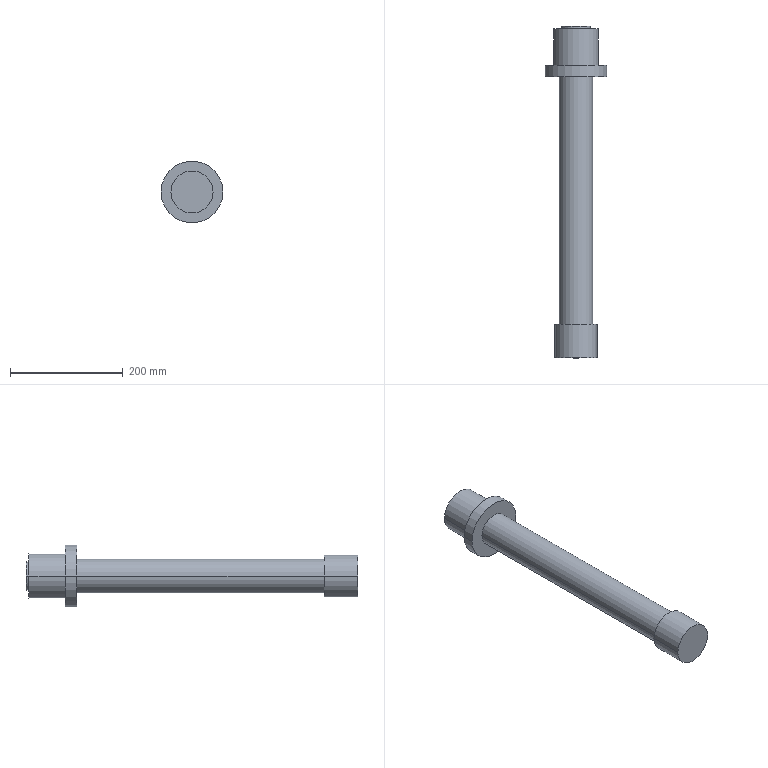Component | SolidWorks | BalanceCylinderBody-1 | 1 solid | 19 faces | box 110 x 590 x 110 mm | volume 957927 mm3 | cylinder 12 | plane 7 | commonest cylinder face diameters 50 x2 51 x2 75 x2 60 x2 110 x2 79 x2
build123d program:
from build123d import *

# Parameters (mm, degrees)
SKETCH2_R           = 25
CUT_EXTRUDE1_DEPTH  = 540
BOSS_EXTRUDE1_START = 5
SKETCH3_R           = 25.5
SKETCH3_R_2         = 25
BOSS_EXTRUDE1_DEPTH = 5


with BuildPart() as part:
    # Sketch1 → Revolve1 (revolve)
    with BuildSketch(Plane(origin=(0, 0, 0), x_dir=(1, 0, 0), z_dir=(0, 1, 0))):
        Polygon((0, 585), (39.5, 585), (39.5, 520), (55, 520), (55, 500), (30, 500), (30, 60), (37.5, 60), (37.5, 0), (0, 0), align=None)
    revolve(axis=Axis((0, 0, 0), (0, 0, -1)))

    # Sketch2 → Cut-Extrude1 (cut)
    with BuildSketch(Plane(origin=(0, 0, -585), x_dir=(-1, 0, 0), z_dir=(0, 0, -1))):
        Circle(SKETCH2_R)
    extrude(amount=-CUT_EXTRUDE1_DEPTH, mode=Mode.SUBTRACT)

    # Sketch3 → Boss-Extrude1 (add)
    with BuildSketch(Plane(origin=(0, 0, -585), x_dir=(-1, 0, 0), z_dir=(0, 0, -1)).offset(BOSS_EXTRUDE1_START)):
        Circle(SKETCH3_R)
        Circle(SKETCH3_R_2, mode=Mode.SUBTRACT)
    extrude(amount=-BOSS_EXTRUDE1_DEPTH)


solid = part.part

# Placed as in the assembly
solid = solid.moved(Location((-101.681, 328.438, 683.723), (90, 0, 0)))
STEP:
#1=CARTESIAN_POINT('',(-3.019,14.702,26.918));
#2=VERTEX_POINT('',#1);
#3=CARTESIAN_POINT('',(-4.987,14.702,26.918));
#4=VERTEX_POINT('',#3);
#5=CARTESIAN_POINT('',(-4.003,14.702,26.918));
#6=DIRECTION('',(0.,1.,0.));
#7=DIRECTION('',(-1.,0.,0.));
#8=AXIS2_PLACEMENT_3D('',#5,#6,#7);
#9=CIRCLE('',#8,0.9843);
#10=EDGE_CURVE('',#2,#4,#9,.T.);
#11=ORIENTED_EDGE('',*,*,#10,.F.);
#12=CARTESIAN_POINT('',(-3.019,36.159,26.918));
#13=VERTEX_POINT('',#12);
#14=CARTESIAN_POINT('',(-3.019,14.702,26.918));
#15=DIRECTION('',(0.,1.,0.));
#16=VECTOR('',#15,39.37);
#17=LINE('',#14,#16);
#18=EDGE_CURVE('',#2,#13,#17,.T.);
#19=ORIENTED_EDGE('',*,*,#18,.T.);
#20=CARTESIAN_POINT('',(-4.987,36.159,26.918));
#21=VERTEX_POINT('',#20);
#22=CARTESIAN_POINT('',(-4.003,36.159,26.918));
#23=DIRECTION('',(0.,1.,0.));
#24=DIRECTION('',(-1.,0.,0.));
#25=AXIS2_PLACEMENT_3D('',#22,#23,#24);
#26=CIRCLE('',#25,0.9843);
#27=EDGE_CURVE('',#13,#21,#26,.T.);
#28=ORIENTED_EDGE('',*,*,#27,.T.);
#29=CARTESIAN_POINT('',(-4.987,14.702,26.918));
#30=DIRECTION('',(0.,1.,0.));
#31=VECTOR('',#30,39.37);
#32=LINE('',#29,#31);
#33=EDGE_CURVE('',#4,#21,#32,.T.);
#34=ORIENTED_EDGE('',*,*,#33,.F.);
#35=EDGE_LOOP('',(#11,#19,#28,#34));
#36=FACE_OUTER_BOUND('',#35,.T.);
#37=CARTESIAN_POINT('',(-4.003,14.702,26.918));
#38=DIRECTION('',(0.,1.,0.));
#39=DIRECTION('',(-1.,0.,0.));
#40=AXIS2_PLACEMENT_3D('',#37,#38,#39);
#41=CYLINDRICAL_SURFACE('',#40,0.9843);
#42=ADVANCED_FACE('',(#36),#41,.F.);
#43=CARTESIAN_POINT('',(-5.007,36.159,26.918));
#44=VERTEX_POINT('',#43);
#45=CARTESIAN_POINT('',(-2.999,36.159,26.918));
#46=VERTEX_POINT('',#45);
#47=CARTESIAN_POINT('',(-4.003,36.159,26.918));
#48=DIRECTION('',(0.,1.,0.));
#49=DIRECTION('',(-1.,0.,0.));
#50=AXIS2_PLACEMENT_3D('',#47,#48,#49);
#51=CIRCLE('',#50,1.004);
#52=EDGE_CURVE('',#44,#46,#51,.T.);
#53=ORIENTED_EDGE('',*,*,#52,.F.);
#54=CARTESIAN_POINT('',(-5.007,35.962,26.918));
#55=VERTEX_POINT('',#54);
#56=CARTESIAN_POINT('',(-5.007,36.159,26.918));
#57=DIRECTION('',(0.,-1.,0.));
#58=VECTOR('',#57,39.37);
#59=LINE('',#56,#58);
#60=EDGE_CURVE('',#44,#55,#59,.T.);
#61=ORIENTED_EDGE('',*,*,#60,.T.);
#62=CARTESIAN_POINT('',(-2.999,35.962,26.918));
#63=VERTEX_POINT('',#62);
#64=CARTESIAN_POINT('',(-4.003,35.962,26.918));
#65=DIRECTION('',(0.,1.,0.));
#66=DIRECTION('',(-1.,0.,0.));
#67=AXIS2_PLACEMENT_3D('',#64,#65,#66);
#68=CIRCLE('',#67,1.004);
#69=EDGE_CURVE('',#55,#63,#68,.T.);
#70=ORIENTED_EDGE('',*,*,#69,.T.);
#71=CARTESIAN_POINT('',(-2.999,36.159,26.918));
#72=DIRECTION('',(0.,-1.,0.));
#73=VECTOR('',#72,39.37);
#74=LINE('',#71,#73);
#75=EDGE_CURVE('',#46,#63,#74,.T.);
#76=ORIENTED_EDGE('',*,*,#75,.F.);
#77=EDGE_LOOP('',(#53,#61,#70,#76));
#78=FACE_OUTER_BOUND('',#77,.T.);
#79=CARTESIAN_POINT('',(-4.003,36.159,26.918));
#80=DIRECTION('',(0.,-1.,0.));
#81=DIRECTION('',(1.,0.,0.));
#82=AXIS2_PLACEMENT_3D('',#79,#80,#81);
#83=CYLINDRICAL_SURFACE('',#82,1.004);
#84=ADVANCED_FACE('',(#78),#83,.T.);
#85=CARTESIAN_POINT('',(-2.527,15.293,26.918));
#86=VERTEX_POINT('',#85);
#87=CARTESIAN_POINT('',(-5.48,15.293,26.918));
#88=VERTEX_POINT('',#87);
#89=CARTESIAN_POINT('',(-4.003,15.293,26.918));
#90=DIRECTION('',(0.,-1.,0.));
#91=DIRECTION('',(1.,0.,0.));
#92=AXIS2_PLACEMENT_3D('',#89,#90,#91);
#93=CIRCLE('',#92,1.476);
#94=EDGE_CURVE('',#86,#88,#93,.T.);
#95=ORIENTED_EDGE('',*,*,#94,.T.);
#96=CARTESIAN_POINT('',(-5.48,12.931,26.918));
#97=VERTEX_POINT('',#96);
#98=CARTESIAN_POINT('',(-5.48,12.931,26.918));
#99=DIRECTION('',(0.,-1.,0.));
#100=VECTOR('',#99,39.37);
#101=LINE('',#98,#100);
#102=EDGE_CURVE('',#88,#97,#101,.T.);
#103=ORIENTED_EDGE('',*,*,#102,.T.);
#104=CARTESIAN_POINT('',(-2.527,12.931,26.918));
#105=VERTEX_POINT('',#104);
#106=CARTESIAN_POINT('',(-4.003,12.931,26.918));
#107=DIRECTION('',(0.,-1.,0.));
#108=DIRECTION('',(1.,0.,0.));
#109=AXIS2_PLACEMENT_3D('',#106,#107,#108);
#110=CIRCLE('',#109,1.476);
#111=EDGE_CURVE('',#105,#97,#110,.T.);
#112=ORIENTED_EDGE('',*,*,#111,.F.);
#113=CARTESIAN_POINT('',(-2.527,12.931,26.918));
#114=DIRECTION('',(0.,-1.,0.));
#115=VECTOR('',#114,39.37);
#116=LINE('',#113,#115);
#117=EDGE_CURVE('',#86,#105,#116,.T.);
#118=ORIENTED_EDGE('',*,*,#117,.F.);
#119=EDGE_LOOP('',(#95,#103,#112,#118));
#120=FACE_OUTER_BOUND('',#119,.T.);
#121=CARTESIAN_POINT('',(-4.003,12.931,26.918));
#122=DIRECTION('',(0.,-1.,0.));
#123=DIRECTION('',(1.,0.,0.));
#124=AXIS2_PLACEMENT_3D('',#121,#122,#123);
#125=CYLINDRICAL_SURFACE('',#124,1.476);
#126=ADVANCED_FACE('',(#120),#125,.T.);
#127=CARTESIAN_POINT('',(-2.822,32.616,26.918));
#128=VERTEX_POINT('',#127);
#129=CARTESIAN_POINT('',(-5.184,32.616,26.918));
#130=VERTEX_POINT('',#129);
#131=CARTESIAN_POINT('',(-4.003,32.616,26.918));
#132=DIRECTION('',(0.,-1.,0.));
#133=DIRECTION('',(1.,0.,0.));
#134=AXIS2_PLACEMENT_3D('',#131,#132,#133);
#135=CIRCLE('',#134,1.181);
#136=EDGE_CURVE('',#128,#130,#135,.T.);
#137=ORIENTED_EDGE('',*,*,#136,.T.);
#138=CARTESIAN_POINT('',(-5.184,15.293,26.918));
#139=VERTEX_POINT('',#138);
#140=CARTESIAN_POINT('',(-5.184,12.931,26.918));
#141=DIRECTION('',(0.,-1.,0.));
#142=VECTOR('',#141,39.37);
#143=LINE('',#140,#142);
#144=EDGE_CURVE('',#130,#139,#143,.T.);
#145=ORIENTED_EDGE('',*,*,#144,.T.);
#146=CARTESIAN_POINT('',(-2.822,15.293,26.918));
#147=VERTEX_POINT('',#146);
#148=CARTESIAN_POINT('',(-4.003,15.293,26.918));
#149=DIRECTION('',(0.,-1.,0.));
#150=DIRECTION('',(1.,0.,0.));
#151=AXIS2_PLACEMENT_3D('',#148,#149,#150);
#152=CIRCLE('',#151,1.181);
#153=EDGE_CURVE('',#147,#139,#152,.T.);
#154=ORIENTED_EDGE('',*,*,#153,.F.);
#155=CARTESIAN_POINT('',(-2.822,12.931,26.918));
#156=DIRECTION('',(0.,-1.,0.));
#157=VECTOR('',#156,39.37);
#158=LINE('',#155,#157);
#159=EDGE_CURVE('',#128,#147,#158,.T.);
#160=ORIENTED_EDGE('',*,*,#159,.F.);
#161=EDGE_LOOP('',(#137,#145,#154,#160));
#162=FACE_OUTER_BOUND('',#161,.T.);
#163=CARTESIAN_POINT('',(-4.003,12.931,26.918));
#164=DIRECTION('',(0.,-1.,0.));
#165=DIRECTION('',(1.,0.,0.));
#166=AXIS2_PLACEMENT_3D('',#163,#164,#165);
#167=CYLINDRICAL_SURFACE('',#166,1.181);
#168=ADVANCED_FACE('',(#162),#167,.T.);
#169=CARTESIAN_POINT('',(-1.838,33.403,26.918));
#170=VERTEX_POINT('',#169);
#171=CARTESIAN_POINT('',(-6.169,33.403,26.918));
#172=VERTEX_POINT('',#171);
#173=CARTESIAN_POINT('',(-4.003,33.403,26.918));
#174=DIRECTION('',(0.,-1.,0.));
#175=DIRECTION('',(1.,0.,0.));
#176=AXIS2_PLACEMENT_3D('',#173,#174,#175);
#177=CIRCLE('',#176,2.165);
#178=EDGE_CURVE('',#170,#172,#177,.T.);
#179=ORIENTED_EDGE('',*,*,#178,.T.);
#180=CARTESIAN_POINT('',(-6.169,32.616,26.918));
#181=VERTEX_POINT('',#180);
#182=CARTESIAN_POINT('',(-6.169,12.931,26.918));
#183=DIRECTION('',(0.,-1.,0.));
#184=VECTOR('',#183,39.37);
#185=LINE('',#182,#184);
#186=EDGE_CURVE('',#172,#181,#185,.T.);
#187=ORIENTED_EDGE('',*,*,#186,.T.);
#188=CARTESIAN_POINT('',(-1.838,32.616,26.918));
#189=VERTEX_POINT('',#188);
#190=CARTESIAN_POINT('',(-4.003,32.616,26.918));
#191=DIRECTION('',(0.,-1.,0.));
#192=DIRECTION('',(1.,0.,0.));
#193=AXIS2_PLACEMENT_3D('',#190,#191,#192);
#194=CIRCLE('',#193,2.165);
#195=EDGE_CURVE('',#189,#181,#194,.T.);
#196=ORIENTED_EDGE('',*,*,#195,.F.);
#197=CARTESIAN_POINT('',(-1.838,12.931,26.918));
#198=DIRECTION('',(0.,-1.,0.));
#199=VECTOR('',#198,39.37);
#200=LINE('',#197,#199);
#201=EDGE_CURVE('',#170,#189,#200,.T.);
#202=ORIENTED_EDGE('',*,*,#201,.F.);
#203=EDGE_LOOP('',(#179,#187,#196,#202));
#204=FACE_OUTER_BOUND('',#203,.T.);
#205=CARTESIAN_POINT('',(-4.003,12.931,26.918));
#206=DIRECTION('',(0.,-1.,0.));
#207=DIRECTION('',(1.,0.,0.));
#208=AXIS2_PLACEMENT_3D('',#205,#206,#207);
#209=CYLINDRICAL_SURFACE('',#208,2.165);
#210=ADVANCED_FACE('',(#204),#209,.T.);
#211=CARTESIAN_POINT('',(-2.448,35.962,26.918));
#212=VERTEX_POINT('',#211);
#213=CARTESIAN_POINT('',(-5.558,35.962,26.918));
#214=VERTEX_POINT('',#213);
#215=CARTESIAN_POINT('',(-4.003,35.962,26.918));
#216=DIRECTION('',(0.,-1.,0.));
#217=DIRECTION('',(1.,0.,0.));
#218=AXIS2_PLACEMENT_3D('',#215,#216,#217);
#219=CIRCLE('',#218,1.555);
#220=EDGE_CURVE('',#212,#214,#219,.T.);
#221=ORIENTED_EDGE('',*,*,#220,.T.);
#222=CARTESIAN_POINT('',(-5.558,33.403,26.918));
#223=VERTEX_POINT('',#222);
#224=CARTESIAN_POINT('',(-5.558,12.931,26.918));
#225=DIRECTION('',(0.,-1.,0.));
#226=VECTOR('',#225,39.37);
#227=LINE('',#224,#226);
#228=EDGE_CURVE('',#214,#223,#227,.T.);
#229=ORIENTED_EDGE('',*,*,#228,.T.);
#230=CARTESIAN_POINT('',(-2.448,33.403,26.918));
#231=VERTEX_POINT('',#230);
#232=CARTESIAN_POINT('',(-4.003,33.403,26.918));
#233=DIRECTION('',(0.,-1.,0.));
#234=DIRECTION('',(1.,0.,0.));
#235=AXIS2_PLACEMENT_3D('',#232,#233,#234);
#236=CIRCLE('',#235,1.555);
#237=EDGE_CURVE('',#231,#223,#236,.T.);
#238=ORIENTED_EDGE('',*,*,#237,.F.);
#239=CARTESIAN_POINT('',(-2.448,12.931,26.918));
#240=DIRECTION('',(0.,-1.,0.));
#241=VECTOR('',#240,39.37);
#242=LINE('',#239,#241);
#243=EDGE_CURVE('',#212,#231,#242,.T.);
#244=ORIENTED_EDGE('',*,*,#243,.F.);
#245=EDGE_LOOP('',(#221,#229,#238,#244));
#246=FACE_OUTER_BOUND('',#245,.T.);
#247=CARTESIAN_POINT('',(-4.003,12.931,26.918));
#248=DIRECTION('',(0.,-1.,0.));
#249=DIRECTION('',(1.,0.,0.));
#250=AXIS2_PLACEMENT_3D('',#247,#248,#249);
#251=CYLINDRICAL_SURFACE('',#250,1.555);
#252=ADVANCED_FACE('',(#246),#251,.T.);
#253=ORIENTED_EDGE('',*,*,#220,.F.);
#254=CARTESIAN_POINT('',(-4.003,35.962,26.918));
#255=DIRECTION('',(0.,-1.,0.));
#256=DIRECTION('',(1.,0.,0.));
#257=AXIS2_PLACEMENT_3D('',#254,#255,#256);
#258=CIRCLE('',#257,1.555);
#259=EDGE_CURVE('',#214,#212,#258,.T.);
#260=ORIENTED_EDGE('',*,*,#259,.F.);
#261=EDGE_LOOP('',(#253,#260));
#262=FACE_OUTER_BOUND('',#261,.T.);
#263=CARTESIAN_POINT('',(-4.003,35.962,26.918));
#264=DIRECTION('',(0.,1.,0.));
#265=DIRECTION('',(-1.,0.,0.));
#266=AXIS2_PLACEMENT_3D('',#263,#264,#265);
#267=CIRCLE('',#266,1.004);
#268=EDGE_CURVE('',#63,#55,#267,.T.);
#269=ORIENTED_EDGE('',*,*,#268,.F.);
#270=ORIENTED_EDGE('',*,*,#69,.F.);
#271=EDGE_LOOP('',(#269,#270));
#272=FACE_BOUND('',#271,.T.);
#273=CARTESIAN_POINT('',(-4.003,35.962,26.918));
#274=DIRECTION('',(0.,1.,0.));
#275=DIRECTION('',(-1.,0.,0.));
#276=AXIS2_PLACEMENT_3D('',#273,#274,#275);
#277=PLANE('',#276);
#278=ADVANCED_FACE('',(#262,#272),#277,.T.);
#279=ORIENTED_EDGE('',*,*,#228,.F.);
#280=ORIENTED_EDGE('',*,*,#259,.T.);
#281=ORIENTED_EDGE('',*,*,#243,.T.);
#282=CARTESIAN_POINT('',(-4.003,33.403,26.918));
#283=DIRECTION('',(0.,-1.,0.));
#284=DIRECTION('',(1.,0.,0.));
#285=AXIS2_PLACEMENT_3D('',#282,#283,#284);
#286=CIRCLE('',#285,1.555);
#287=EDGE_CURVE('',#223,#231,#286,.T.);
#288=ORIENTED_EDGE('',*,*,#287,.F.);
#289=EDGE_LOOP('',(#279,#280,#281,#288));
#290=FACE_OUTER_BOUND('',#289,.T.);
#291=CARTESIAN_POINT('',(-4.003,12.931,26.918));
#292=DIRECTION('',(0.,-1.,0.));
#293=DIRECTION('',(1.,0.,0.));
#294=AXIS2_PLACEMENT_3D('',#291,#292,#293);
#295=CYLINDRICAL_SURFACE('',#294,1.555);
#296=ADVANCED_FACE('',(#290),#295,.T.);
#297=ORIENTED_EDGE('',*,*,#237,.T.);
#298=ORIENTED_EDGE('',*,*,#287,.T.);
#299=EDGE_LOOP('',(#297,#298));
#300=FACE_BOUND('',#299,.T.);
#301=ORIENTED_EDGE('',*,*,#178,.F.);
#302=CARTESIAN_POINT('',(-4.003,33.403,26.918));
#303=DIRECTION('',(0.,-1.,0.));
#304=DIRECTION('',(1.,0.,0.));
#305=AXIS2_PLACEMENT_3D('',#302,#303,#304);
#306=CIRCLE('',#305,2.165);
#307=EDGE_CURVE('',#172,#170,#306,.T.);
#308=ORIENTED_EDGE('',*,*,#307,.F.);
#309=EDGE_LOOP('',(#301,#308));
#310=FACE_OUTER_BOUND('',#309,.T.);
#311=CARTESIAN_POINT('',(-2.448,33.403,26.918));
#312=DIRECTION('',(0.,1.,0.));
#313=DIRECTION('',(-1.,0.,0.));
#314=AXIS2_PLACEMENT_3D('',#311,#312,#313);
#315=PLANE('',#314);
#316=ADVANCED_FACE('',(#300,#310),#315,.T.);
#317=ORIENTED_EDGE('',*,*,#186,.F.);
#318=ORIENTED_EDGE('',*,*,#307,.T.);
#319=ORIENTED_EDGE('',*,*,#201,.T.);
#320=CARTESIAN_POINT('',(-4.003,32.616,26.918));
#321=DIRECTION('',(0.,-1.,0.));
#322=DIRECTION('',(1.,0.,0.));
#323=AXIS2_PLACEMENT_3D('',#320,#321,#322);
#324=CIRCLE('',#323,2.165);
#325=EDGE_CURVE('',#181,#189,#324,.T.);
#326=ORIENTED_EDGE('',*,*,#325,.F.);
#327=EDGE_LOOP('',(#317,#318,#319,#326));
#328=FACE_OUTER_BOUND('',#327,.T.);
#329=CARTESIAN_POINT('',(-4.003,12.931,26.918));
#330=DIRECTION('',(0.,-1.,0.));
#331=DIRECTION('',(1.,0.,0.));
#332=AXIS2_PLACEMENT_3D('',#329,#330,#331);
#333=CYLINDRICAL_SURFACE('',#332,2.165);
#334=ADVANCED_FACE('',(#328),#333,.T.);
#335=ORIENTED_EDGE('',*,*,#195,.T.);
#336=ORIENTED_EDGE('',*,*,#325,.T.);
#337=EDGE_LOOP('',(#335,#336));
#338=FACE_OUTER_BOUND('',#337,.T.);
#339=ORIENTED_EDGE('',*,*,#136,.F.);
#340=CARTESIAN_POINT('',(-4.003,32.616,26.918));
#341=DIRECTION('',(0.,-1.,0.));
#342=DIRECTION('',(1.,0.,0.));
#343=AXIS2_PLACEMENT_3D('',#340,#341,#342);
#344=CIRCLE('',#343,1.181);
#345=EDGE_CURVE('',#130,#128,#344,.T.);
#346=ORIENTED_EDGE('',*,*,#345,.F.);
#347=EDGE_LOOP('',(#339,#346));
#348=FACE_BOUND('',#347,.T.);
#349=CARTESIAN_POINT('',(-1.838,32.616,26.918));
#350=DIRECTION('',(0.,-1.,0.));
#351=DIRECTION('',(1.,0.,0.));
#352=AXIS2_PLACEMENT_3D('',#349,#350,#351);
#353=PLANE('',#352);
#354=ADVANCED_FACE('',(#338,#348),#353,.T.);
#355=ORIENTED_EDGE('',*,*,#144,.F.);
#356=ORIENTED_EDGE('',*,*,#345,.T.);
#357=ORIENTED_EDGE('',*,*,#159,.T.);
#358=CARTESIAN_POINT('',(-4.003,15.293,26.918));
#359=DIRECTION('',(0.,-1.,0.));
#360=DIRECTION('',(1.,0.,0.));
#361=AXIS2_PLACEMENT_3D('',#358,#359,#360);
#362=CIRCLE('',#361,1.181);
#363=EDGE_CURVE('',#139,#147,#362,.T.);
#364=ORIENTED_EDGE('',*,*,#363,.F.);
#365=EDGE_LOOP('',(#355,#356,#357,#364));
#366=FACE_OUTER_BOUND('',#365,.T.);
#367=CARTESIAN_POINT('',(-4.003,12.931,26.918));
#368=DIRECTION('',(0.,-1.,0.));
#369=DIRECTION('',(1.,0.,0.));
#370=AXIS2_PLACEMENT_3D('',#367,#368,#369);
#371=CYLINDRICAL_SURFACE('',#370,1.181);
#372=ADVANCED_FACE('',(#366),#371,.T.);
#373=ORIENTED_EDGE('',*,*,#153,.T.);
#374=ORIENTED_EDGE('',*,*,#363,.T.);
#375=EDGE_LOOP('',(#373,#374));
#376=FACE_BOUND('',#375,.T.);
#377=ORIENTED_EDGE('',*,*,#94,.F.);
#378=CARTESIAN_POINT('',(-4.003,15.293,26.918));
#379=DIRECTION('',(0.,-1.,0.));
#380=DIRECTION('',(1.,0.,0.));
#381=AXIS2_PLACEMENT_3D('',#378,#379,#380);
#382=CIRCLE('',#381,1.476);
#383=EDGE_CURVE('',#88,#86,#382,.T.);
#384=ORIENTED_EDGE('',*,*,#383,.F.);
#385=EDGE_LOOP('',(#377,#384));
#386=FACE_OUTER_BOUND('',#385,.T.);
#387=CARTESIAN_POINT('',(-2.822,15.293,26.918));
#388=DIRECTION('',(0.,1.,0.));
#389=DIRECTION('',(-1.,0.,0.));
#390=AXIS2_PLACEMENT_3D('',#387,#388,#389);
#391=PLANE('',#390);
#392=ADVANCED_FACE('',(#376,#386),#391,.T.);
#393=ORIENTED_EDGE('',*,*,#102,.F.);
#394=ORIENTED_EDGE('',*,*,#383,.T.);
#395=ORIENTED_EDGE('',*,*,#117,.T.);
#396=CARTESIAN_POINT('',(-4.003,12.931,26.918));
#397=DIRECTION('',(0.,-1.,0.));
#398=DIRECTION('',(1.,0.,0.));
#399=AXIS2_PLACEMENT_3D('',#396,#397,#398);
#400=CIRCLE('',#399,1.476);
#401=EDGE_CURVE('',#97,#105,#400,.T.);
#402=ORIENTED_EDGE('',*,*,#401,.F.);
#403=EDGE_LOOP('',(#393,#394,#395,#402));
#404=FACE_OUTER_BOUND('',#403,.T.);
#405=CARTESIAN_POINT('',(-4.003,12.931,26.918));
#406=DIRECTION('',(0.,-1.,0.));
#407=DIRECTION('',(1.,0.,0.));
#408=AXIS2_PLACEMENT_3D('',#405,#406,#407);
#409=CYLINDRICAL_SURFACE('',#408,1.476);
#410=ADVANCED_FACE('',(#404),#409,.T.);
#411=ORIENTED_EDGE('',*,*,#111,.T.);
#412=ORIENTED_EDGE('',*,*,#401,.T.);
#413=EDGE_LOOP('',(#411,#412));
#414=FACE_OUTER_BOUND('',#413,.T.);
#415=CARTESIAN_POINT('',(-2.527,12.931,26.918));
#416=DIRECTION('',(0.,-1.,0.));
#417=DIRECTION('',(1.,0.,0.));
#418=AXIS2_PLACEMENT_3D('',#415,#416,#417);
#419=PLANE('',#418);
#420=ADVANCED_FACE('',(#414),#419,.T.);
#421=CARTESIAN_POINT('',(-4.003,36.159,26.918));
#422=DIRECTION('',(0.,1.,0.));
#423=DIRECTION('',(-1.,0.,0.));
#424=AXIS2_PLACEMENT_3D('',#421,#422,#423);
#425=CIRCLE('',#424,1.004);
#426=EDGE_CURVE('',#46,#44,#425,.T.);
#427=ORIENTED_EDGE('',*,*,#426,.T.);
#428=ORIENTED_EDGE('',*,*,#52,.T.);
#429=EDGE_LOOP('',(#427,#428));
#430=FACE_OUTER_BOUND('',#429,.T.);
#431=CARTESIAN_POINT('',(-4.003,36.159,26.918));
#432=DIRECTION('',(0.,1.,0.));
#433=DIRECTION('',(-1.,0.,0.));
#434=AXIS2_PLACEMENT_3D('',#431,#432,#433);
#435=CIRCLE('',#434,0.9843);
#436=EDGE_CURVE('',#21,#13,#435,.T.);
#437=ORIENTED_EDGE('',*,*,#436,.F.);
#438=ORIENTED_EDGE('',*,*,#27,.F.);
#439=EDGE_LOOP('',(#437,#438));
#440=FACE_BOUND('',#439,.T.);
#441=CARTESIAN_POINT('',(-4.003,36.159,26.918));
#442=DIRECTION('',(0.,1.,0.));
#443=DIRECTION('',(-1.,0.,0.));
#444=AXIS2_PLACEMENT_3D('',#441,#442,#443);
#445=PLANE('',#444);
#446=ADVANCED_FACE('',(#430,#440),#445,.T.);
#447=ORIENTED_EDGE('',*,*,#60,.F.);
#448=ORIENTED_EDGE('',*,*,#426,.F.);
#449=ORIENTED_EDGE('',*,*,#75,.T.);
#450=ORIENTED_EDGE('',*,*,#268,.T.);
#451=EDGE_LOOP('',(#447,#448,#449,#450));
#452=FACE_OUTER_BOUND('',#451,.T.);
#453=CARTESIAN_POINT('',(-4.003,36.159,26.918));
#454=DIRECTION('',(0.,-1.,0.));
#455=DIRECTION('',(1.,0.,0.));
#456=AXIS2_PLACEMENT_3D('',#453,#454,#455);
#457=CYLINDRICAL_SURFACE('',#456,1.004);
#458=ADVANCED_FACE('',(#452),#457,.T.);
#459=CARTESIAN_POINT('',(-4.003,14.702,26.918));
#460=DIRECTION('',(0.,1.,0.));
#461=DIRECTION('',(-1.,0.,0.));
#462=AXIS2_PLACEMENT_3D('',#459,#460,#461);
#463=CIRCLE('',#462,0.9843);
#464=EDGE_CURVE('',#4,#2,#463,.T.);
#465=ORIENTED_EDGE('',*,*,#464,.T.);
#466=ORIENTED_EDGE('',*,*,#10,.T.);
#467=EDGE_LOOP('',(#465,#466));
#468=FACE_OUTER_BOUND('',#467,.T.);
#469=CARTESIAN_POINT('',(-4.003,14.702,26.918));
#470=DIRECTION('',(0.,1.,0.));
#471=DIRECTION('',(-1.,0.,0.));
#472=AXIS2_PLACEMENT_3D('',#469,#470,#471);
#473=PLANE('',#472);
#474=ADVANCED_FACE('',(#468),#473,.T.);
#475=ORIENTED_EDGE('',*,*,#18,.F.);
#476=ORIENTED_EDGE('',*,*,#464,.F.);
#477=ORIENTED_EDGE('',*,*,#33,.T.);
#478=ORIENTED_EDGE('',*,*,#436,.T.);
#479=EDGE_LOOP('',(#475,#476,#477,#478));
#480=FACE_OUTER_BOUND('',#479,.T.);
#481=CARTESIAN_POINT('',(-4.003,14.702,26.918));
#482=DIRECTION('',(0.,1.,0.));
#483=DIRECTION('',(-1.,0.,0.));
#484=AXIS2_PLACEMENT_3D('',#481,#482,#483);
#485=CYLINDRICAL_SURFACE('',#484,0.9843);
#486=ADVANCED_FACE('',(#480),#485,.F.);
#487=CLOSED_SHELL('',(#42,#84,#126,#168,#210,#252,#278,#296,#316,#334,#354,#372,#392,#410,#420,#446,#458,#474,#486));
#488=MANIFOLD_SOLID_BREP('',#487);
#489=CARTESIAN_POINT('',(0.,0.,0.));
#490=DIRECTION('',(0.,0.,1.));
#491=DIRECTION('',(1.,0.,0.));
#492=AXIS2_PLACEMENT_3D('',#489,#490,#491);
#493=(LENGTH_UNIT()NAMED_UNIT(*)SI_UNIT($,.METRE.));
#494=LENGTH_MEASURE_WITH_UNIT(LENGTH_MEASURE(0.0254),#493);
#495=DIMENSIONAL_EXPONENTS(1.,0.,0.,0.,0.,0.,0.);
#496=(CONVERSION_BASED_UNIT('',#494)LENGTH_UNIT()NAMED_UNIT(#495));
#497=UNCERTAINTY_MEASURE_WITH_UNIT(LENGTH_MEASURE(0.00001),#496,'','');
#498=(NAMED_UNIT(*)PLANE_ANGLE_UNIT()SI_UNIT($,.RADIAN.));
#499=(NAMED_UNIT(*)SI_UNIT($,.STERADIAN.)SOLID_ANGLE_UNIT());
#500=(GEOMETRIC_REPRESENTATION_CONTEXT(3)GLOBAL_UNCERTAINTY_ASSIGNED_CONTEXT((#497))GLOBAL_UNIT_ASSIGNED_CONTEXT((#496,#498,#499))REPRESENTATION_CONTEXT('',''));
#501=ADVANCED_BREP_SHAPE_REPRESENTATION('',(#488,#492),#500);
#502=COLOUR_RGB('',0.7922,0.8196,0.9333);
#503=FILL_AREA_STYLE_COLOUR('',#502);
#504=FILL_AREA_STYLE('',(#503));
#505=SURFACE_STYLE_FILL_AREA(#504);
#506=SURFACE_SIDE_STYLE('',(#505));
#507=SURFACE_STYLE_USAGE(.BOTH.,#506);
#508=PRESENTATION_STYLE_ASSIGNMENT((#507));
#509=STYLED_ITEM('',(#508),#488);
#510=(LENGTH_UNIT()NAMED_UNIT(*)SI_UNIT($,.METRE.));
#511=LENGTH_MEASURE_WITH_UNIT(LENGTH_MEASURE(0.0254),#510);
#512=DIMENSIONAL_EXPONENTS(1.,0.,0.,0.,0.,0.,0.);
#513=(CONVERSION_BASED_UNIT('',#511)LENGTH_UNIT()NAMED_UNIT(#512));
#514=UNCERTAINTY_MEASURE_WITH_UNIT(LENGTH_MEASURE(0.00001),#513,'','');
#515=(NAMED_UNIT(*)PLANE_ANGLE_UNIT()SI_UNIT($,.RADIAN.));
#516=(NAMED_UNIT(*)SI_UNIT($,.STERADIAN.)SOLID_ANGLE_UNIT());
#517=(GEOMETRIC_REPRESENTATION_CONTEXT(3)GLOBAL_UNCERTAINTY_ASSIGNED_CONTEXT((#514))GLOBAL_UNIT_ASSIGNED_CONTEXT((#513,#515,#516))REPRESENTATION_CONTEXT('',''));
#518=MECHANICAL_DESIGN_GEOMETRIC_PRESENTATION_REPRESENTATION('',(#509),#517);
#519=PRESENTATION_LAYER_ASSIGNMENT('','',(#509));